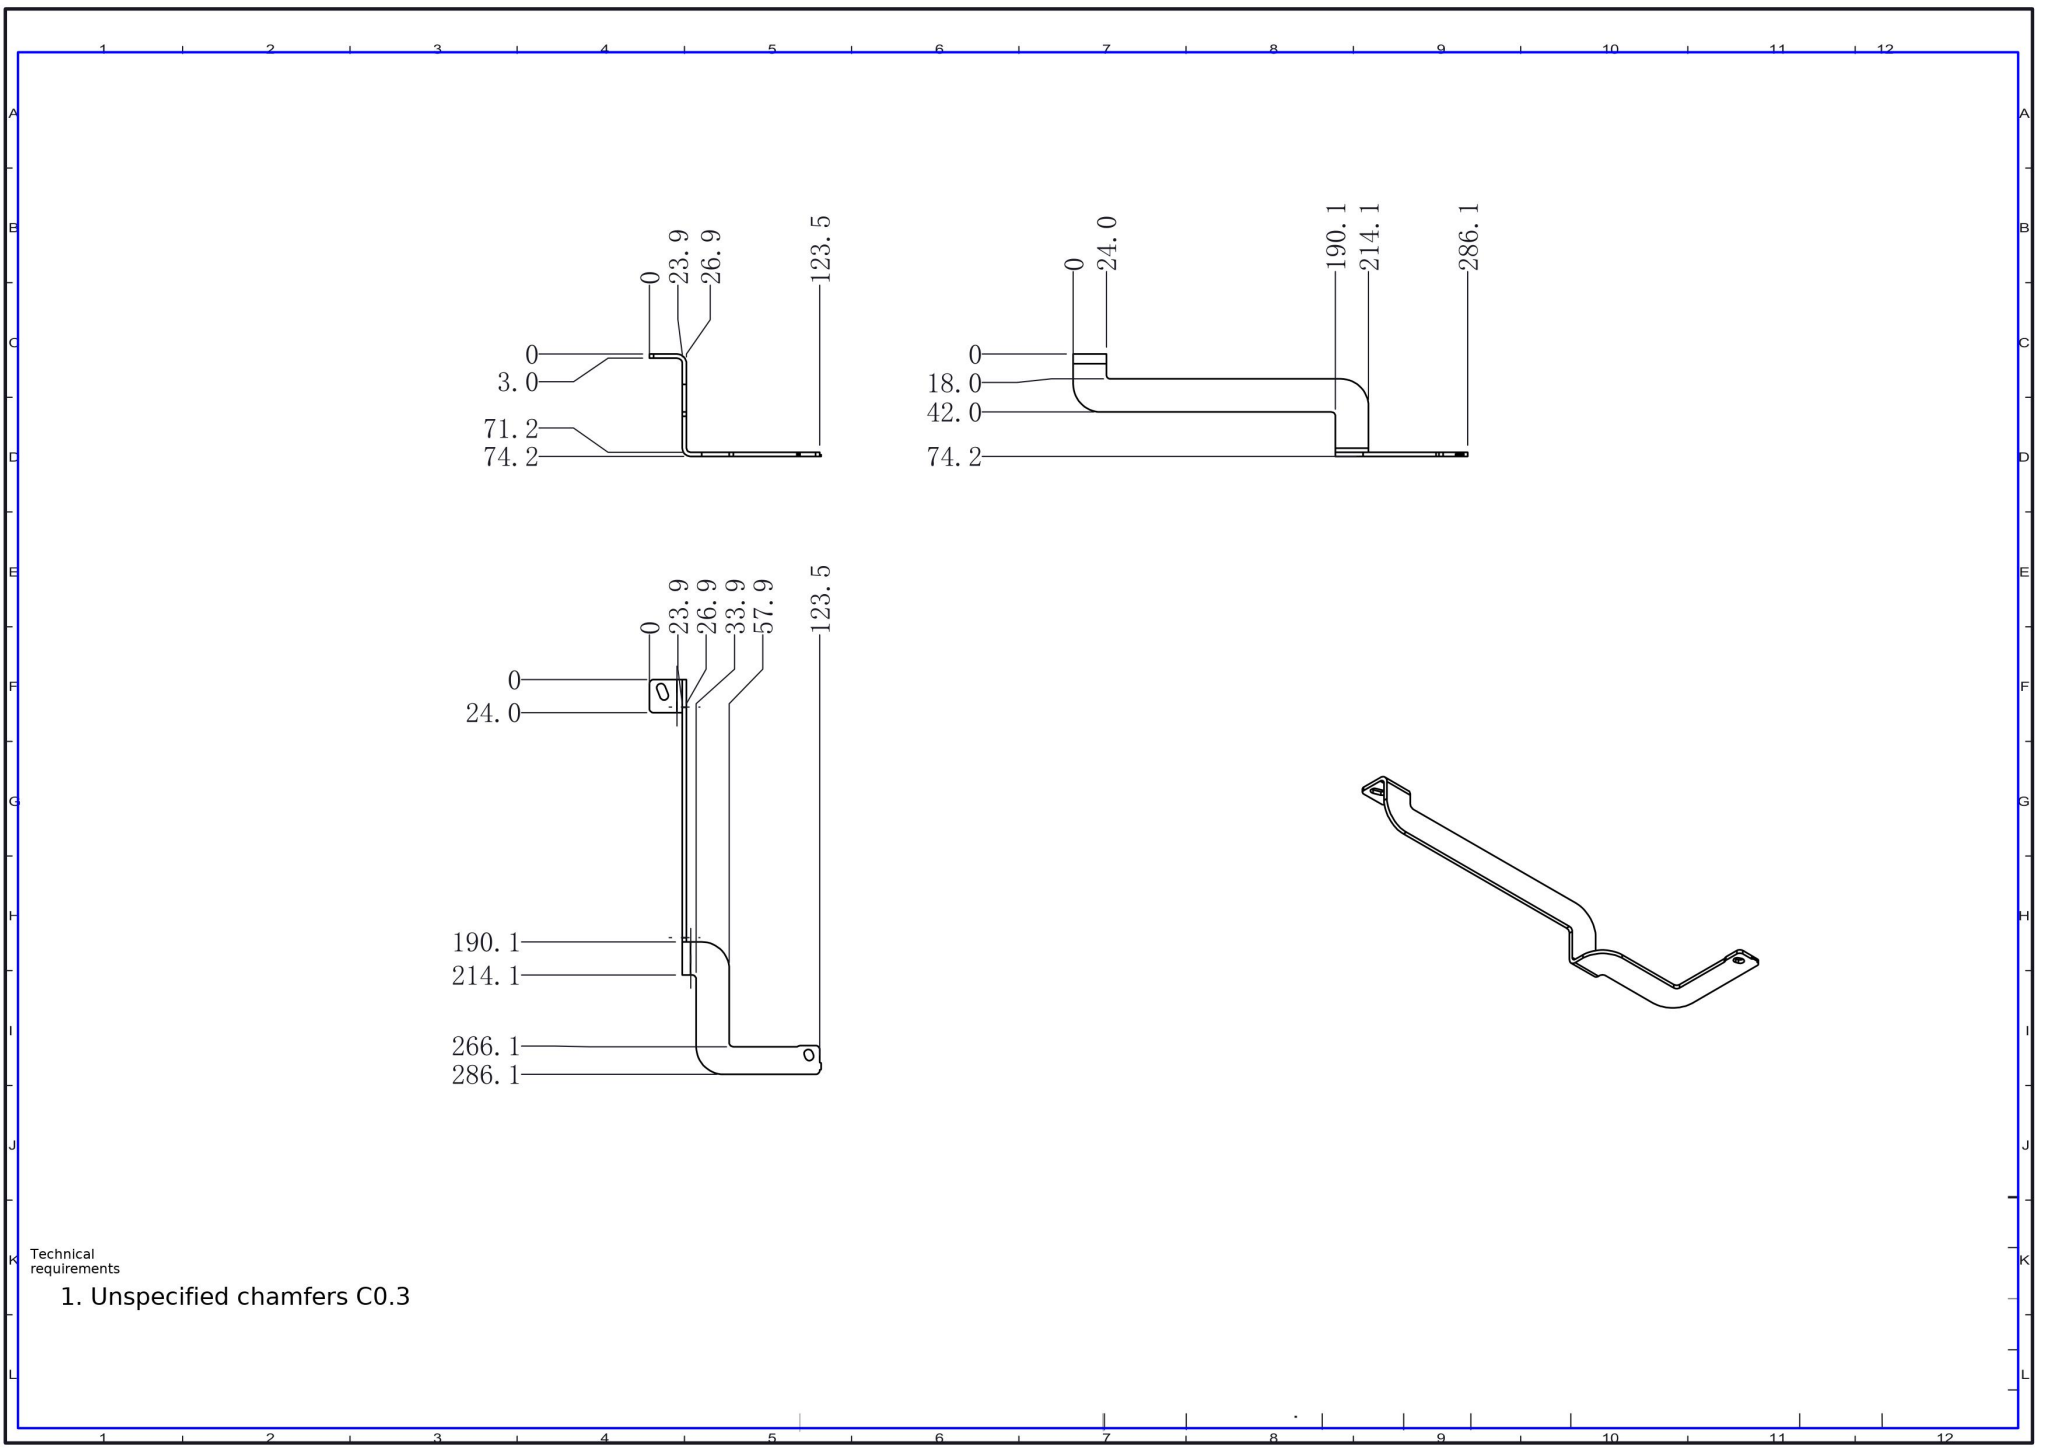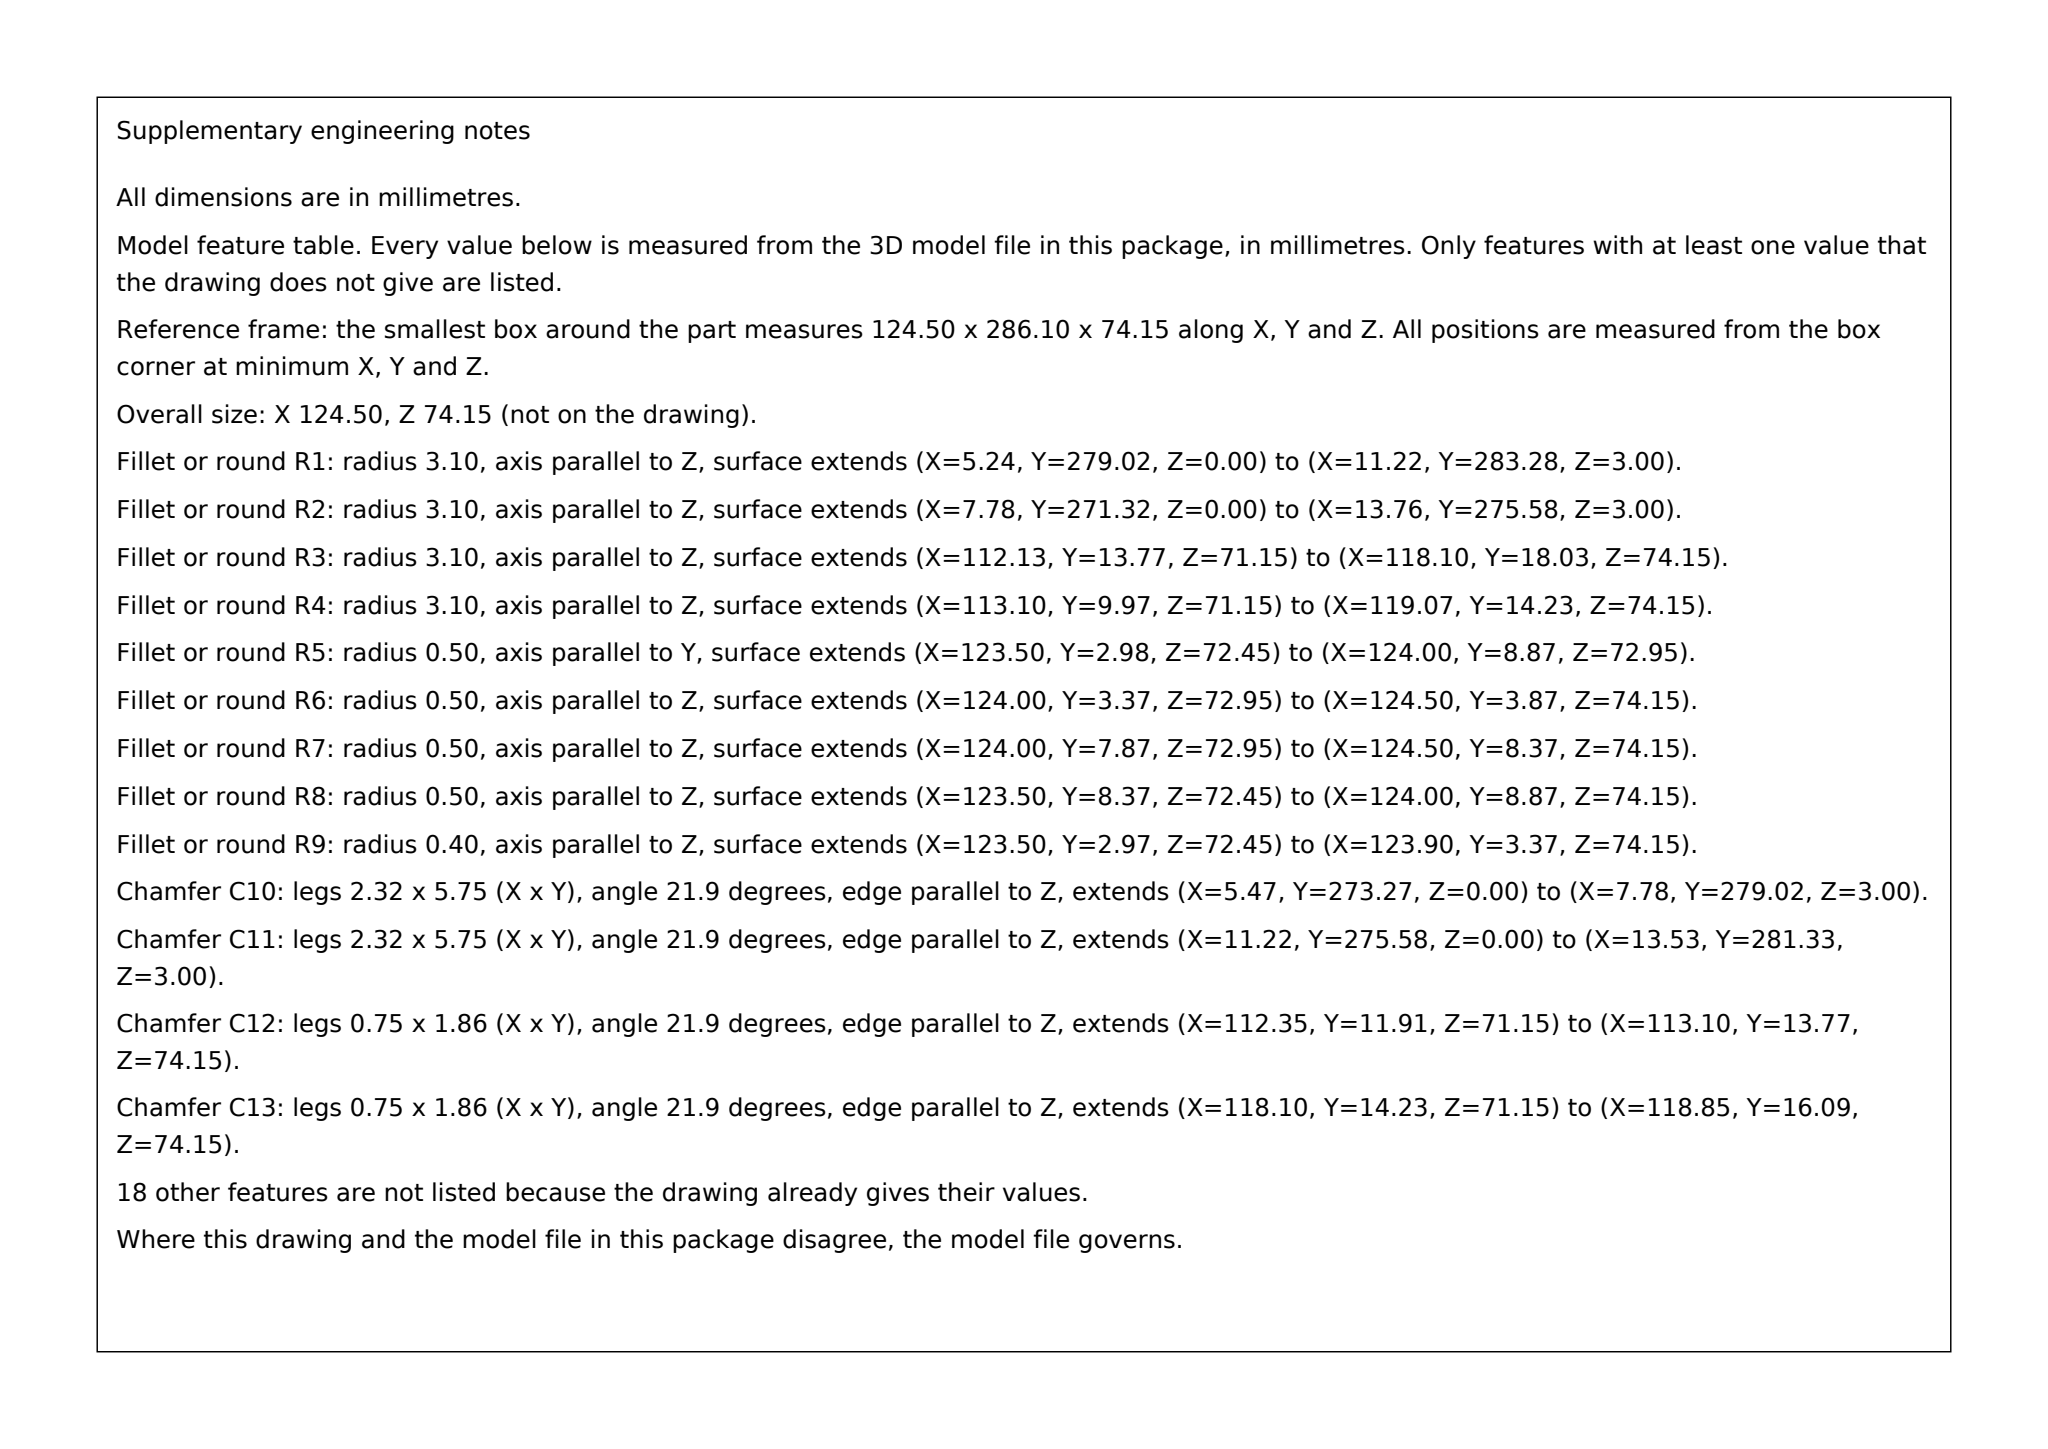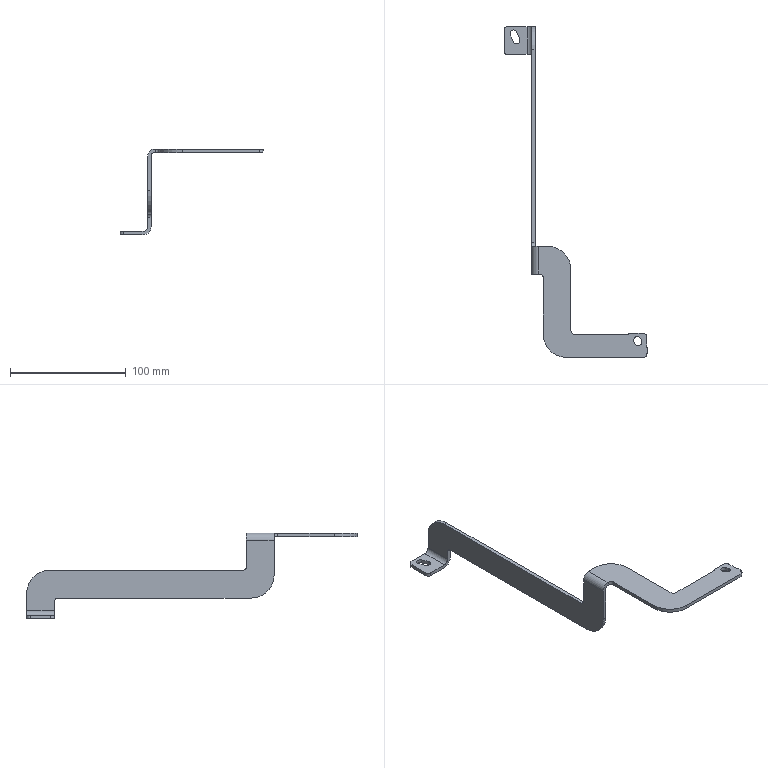Part | SolidWorks | mm | 1 solid | 55 faces | box 124.5 x 286.1 x 74.15 mm | volume 30471 mm3 | cylinder 29 | plane 26 | commonest cylinder face diameters 6 x9 6.2 x6 40 x4 1 x4 4 x2 14 x1 12 x1 8 x1